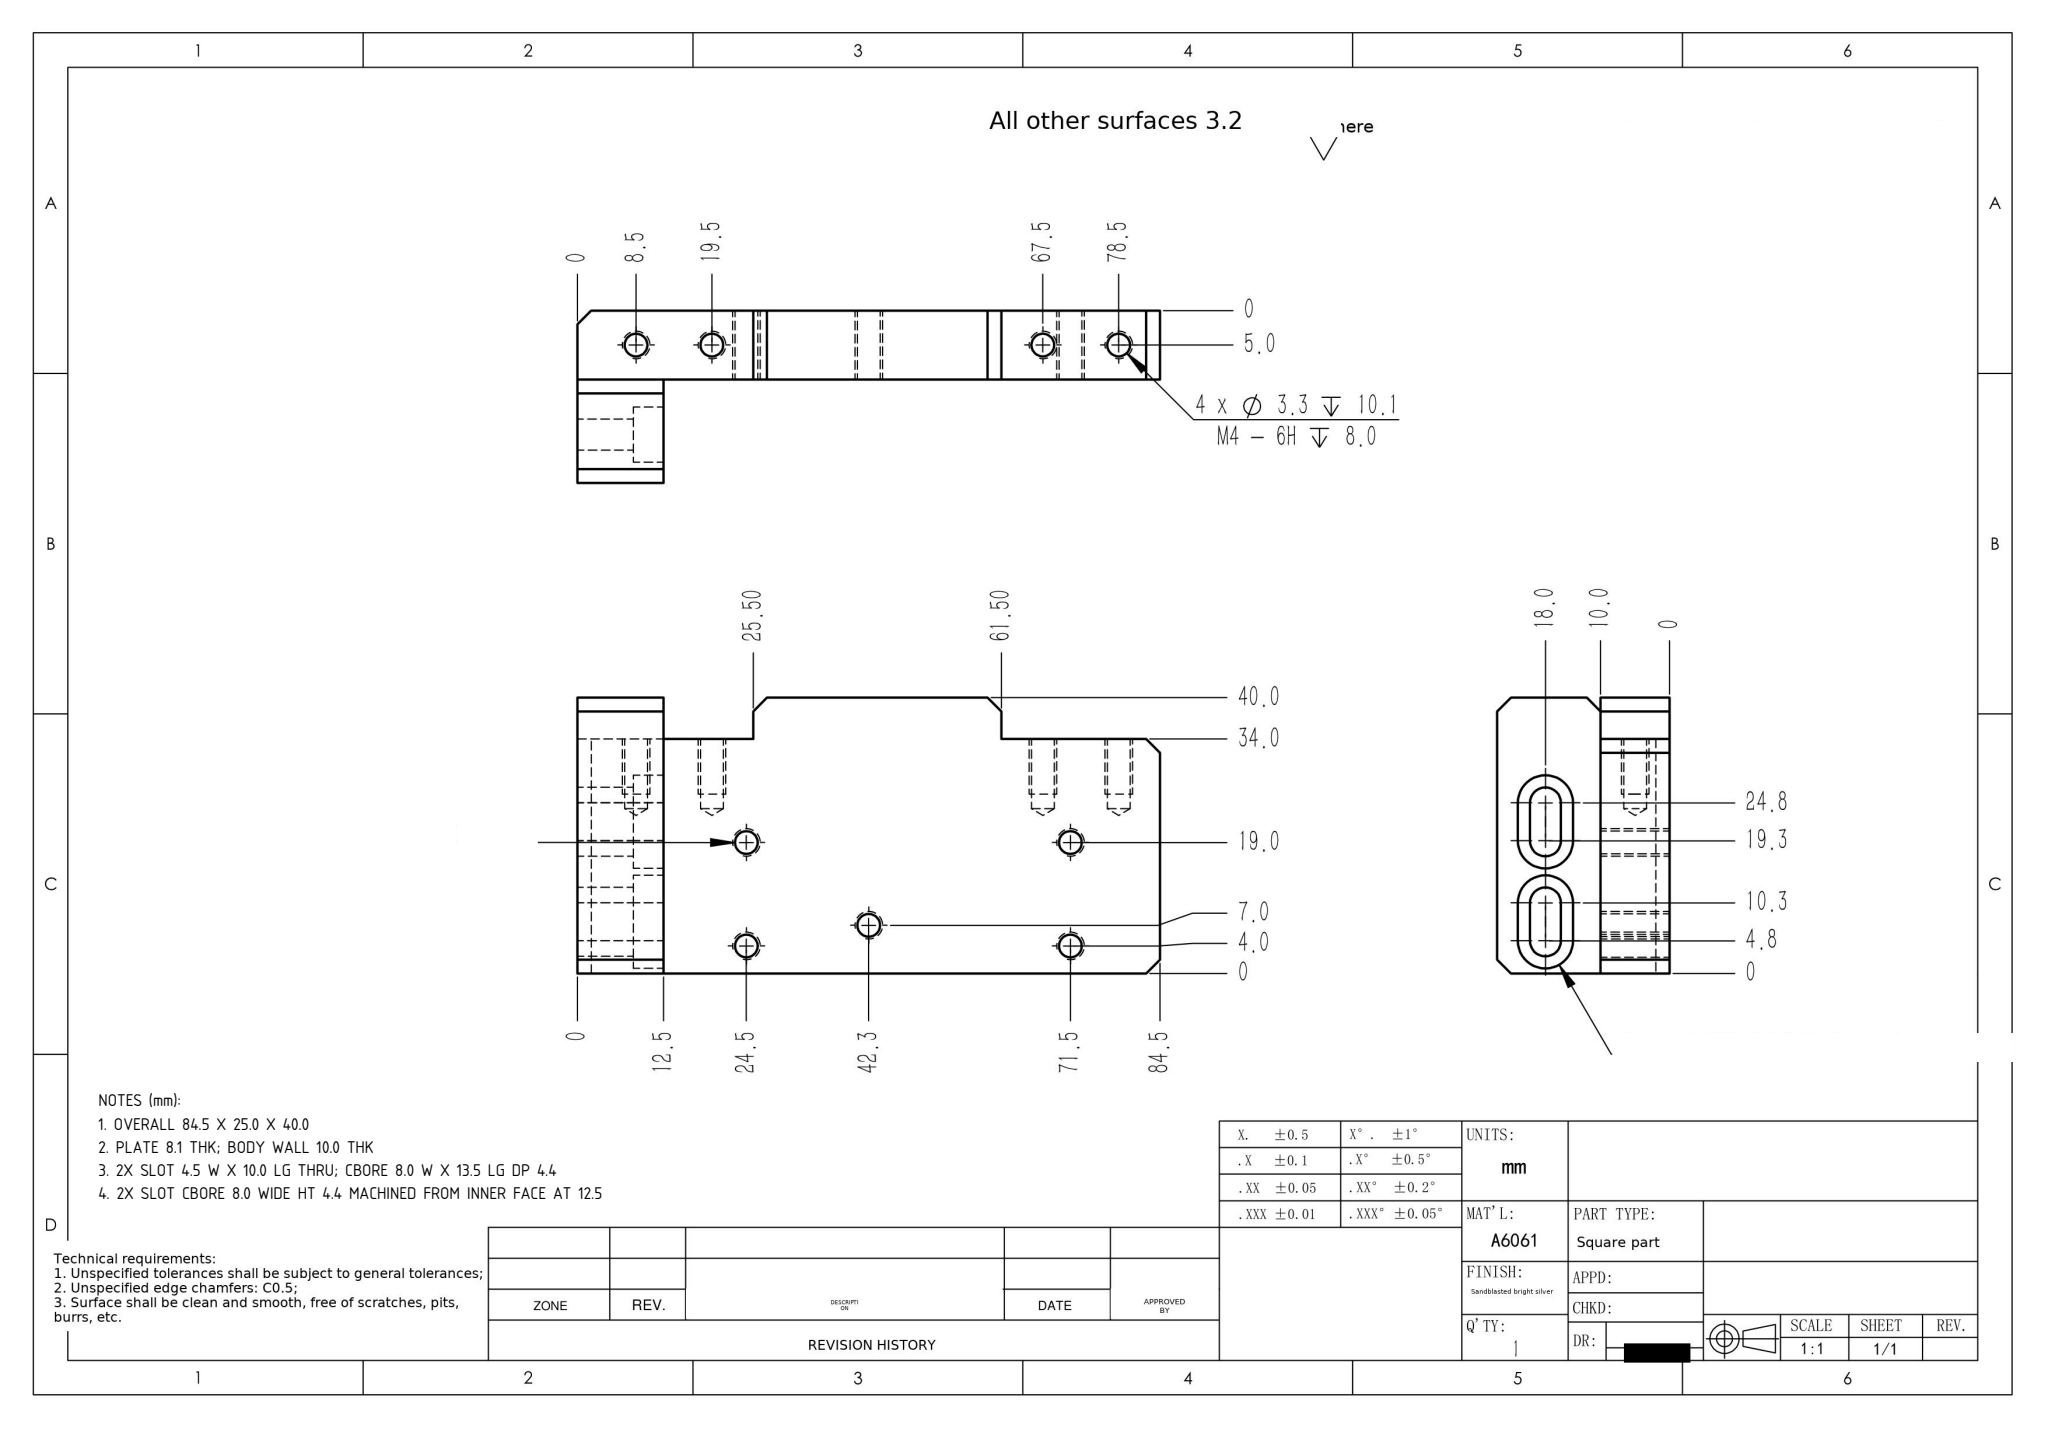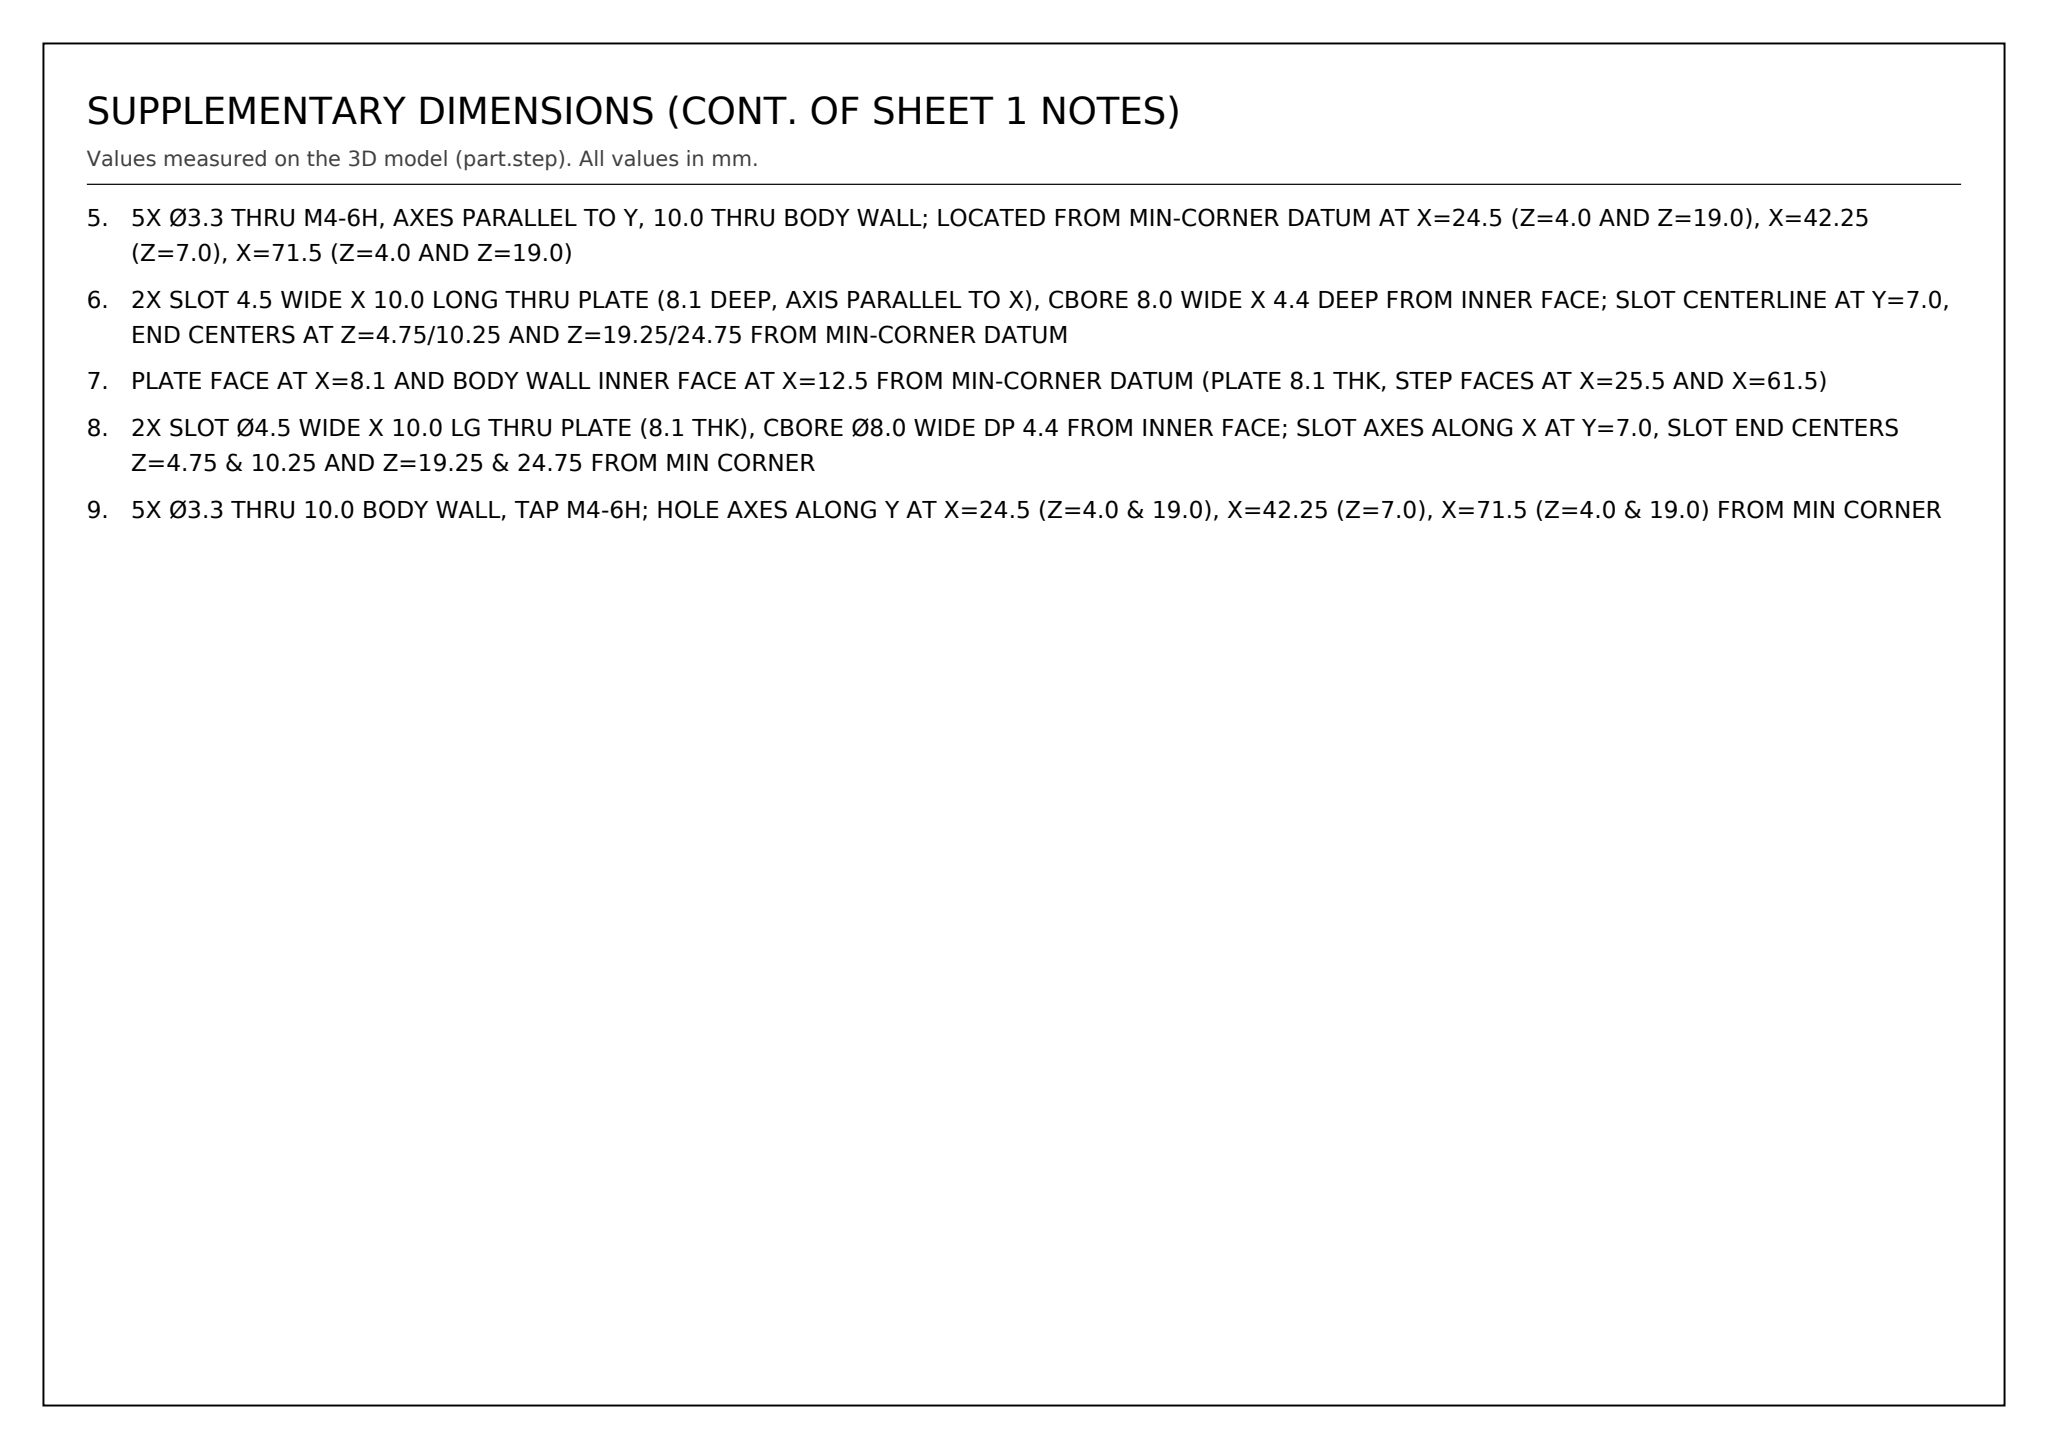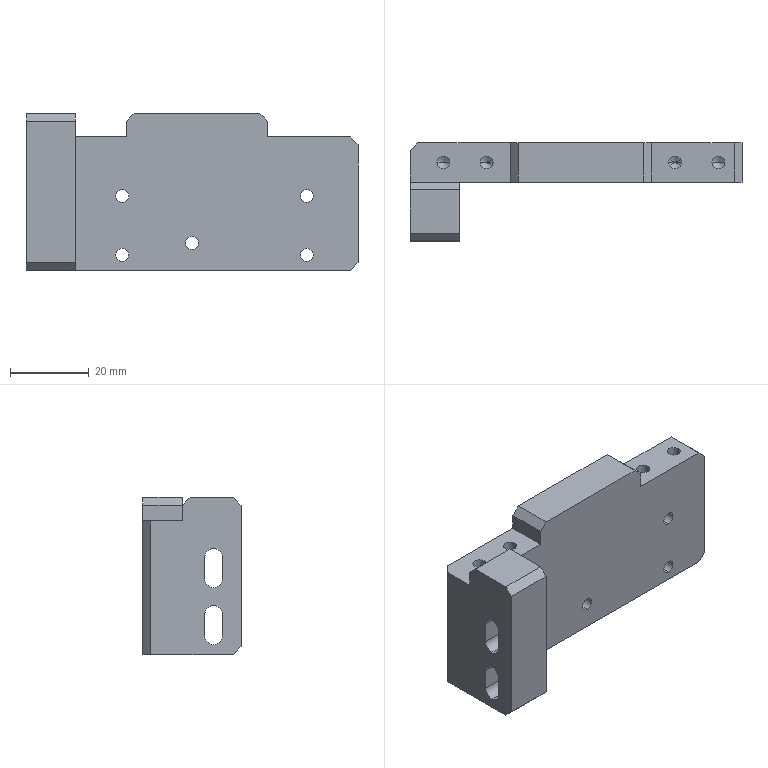Part | SolidWorks | mm | 1 solid | 70 faces | box 84.5 x 25 x 40 mm | volume 35894 mm3 | plane 32 | cylinder 30 | cone 8 | commonest cylinder face diameters 3.3 x18 8 x6 4.5 x6
Drawing notes:
OVERALL 84.5 X 25.0 X 40.0 | from the solid: bbox_xyz [84.5, 25.0, 40.0]
PLATE 8.1 THK; BODY WALL 10.0 THK | from the solid: x planes 0.0 & 8.1 = plate thk; y planes 15.0 & 25.0 with O3.3 y-holes L=10.0 = wall
2X SLOT 4.5 W X 10.0 LG THRU; CBORE 8.0 W X 13.5 LG DP 4.4 | from the solid: O4.5 x-axis cyls L=8.1 at z=4.75/10.25 & 19.25/24.75 (y=7.0); O8.0 x-axis cyls L=4.4 same CLs
2X SLOT CBORE 8.0 WIDE HT 4.4 MACHINED FROM INNER FACE AT 12.5 | from the solid: Dia 8.0 x-axis cbores (len 4.4) run from x=12.5 face to plane x=8.1; 4.5 dia (len 8.1) continues to x=0, so cbore opens on the x=12.5 face of the 12.5 thk plate
5X Ø3.3 THRU M4-6H, AXES PARALLEL TO Y, 10.0 THRU BODY WALL; LOCATED FROM MIN-CORNER DATUM AT X=24.5 (Z=4.0 AND Z=19.0), X=42.25 (Z=7.0), X=71.5 (Z=4.0 AND Z=19.0) | from the solid: cylinders dia 3.3 axis y at [24.5,-,4.0], [24.5,-,19.0], [42.25,-,7.0], [71.5,-,4.0], [71.5,-,19.0], length 10.0
2X SLOT 4.5 WIDE X 10.0 LONG THRU PLATE (8.1 DEEP, AXIS PARALLEL TO X), CBORE 8.0 WIDE X 4.4 DEEP FROM INNER FACE; SLOT CENTERLINE AT Y=7.0, END CENTERS AT Z=4.75/10.25 AND Z=19.25/24.75 FROM MIN-CORNER DATUM | from the solid: cylinders dia 4.5 axis x at y=7.0, z=4.75/10.25/19.25/24.75, length 8.1; cylinders dia 8.0 axis x same positions, length 4.4
PLATE FACE AT X=8.1 AND BODY WALL INNER FACE AT X=12.5 FROM MIN-CORNER DATUM (PLATE 8.1 THK, STEP FACES AT X=25.5 AND X=61.5) | from the solid: axis_planes x = 0.0, 8.1, 12.5, 25.5, 61.5, 84.5
2X SLOT Ø4.5 WIDE X 10.0 LG THRU PLATE (8.1 THK), CBORE Ø8.0 WIDE DP 4.4 FROM INNER FACE; SLOT AXES ALONG X AT Y=7.0, SLOT END CENTERS Z=4.75 & 10.25 AND Z=19.25 & 24.75 FROM MIN CORNER | from the solid: cylinders dia 4.5 axis x len 8.1 at [y=7.0, z=4.75/10.25/19.25/24.75] and dia 8.0 axis x len 4.4 at same positions; plane x=8.1
5X Ø3.3 THRU 10.0 BODY WALL, TAP M4-6H; HOLE AXES ALONG Y AT X=24.5 (Z=4.0 & 19.0), X=42.25 (Z=7.0), X=71.5 (Z=4.0 & 19.0) FROM MIN CORNER | from the solid: cylinders dia 3.3 axis y len 10.0 at [24.5,4.0], [24.5,19.0], [42.25,7.0], [71.5,4.0], [71.5,19.0]; planes y=15.0 and y=25.0